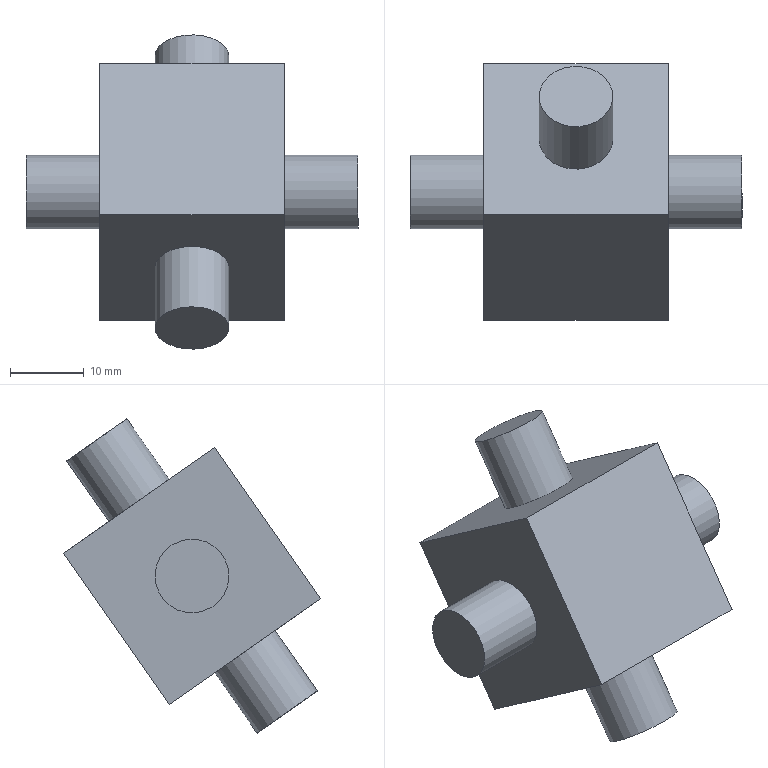Component | NX | UNIVERSAL_JOINT_CENTER_BLOCK_MODEL1 | 1 solid | 14 faces | box 45 x 34.82 x 42.6 mm | volume 18767 mm3 | plane 10 | cylinder 4 | commonest cylinder face diameters 10 x4
STEP:
#1=CARTESIAN_POINT('',(0.,0.,0.));
#2=DIRECTION('',(0.,0.,1.));
#3=DIRECTION('',(1.,0.,0.));
#4=AXIS2_PLACEMENT_3D('',#1,#2,#3);
#5=CARTESIAN_POINT('',(12.5,475.368,-241.274));
#6=VERTEX_POINT('',#5);
#7=CARTESIAN_POINT('',(12.5,461.028,-261.753));
#8=VERTEX_POINT('',#7);
#9=CARTESIAN_POINT('',(12.5,475.368,-241.274));
#10=DIRECTION('',(0.,-0.5736,-0.8192));
#11=VECTOR('',#10,1.);
#12=LINE('',#9,#11);
#13=CARTESIAN_POINT('',(-12.5,475.368,-241.274));
#14=DIRECTION('',(-0.,-0.8192,0.5736));
#15=DIRECTION('',(1.,-0.,0.));
#16=AXIS2_PLACEMENT_3D('',#13,#14,#15);
#17=PLANE('',#16);
#18=CARTESIAN_POINT('',(25.,-0.));
#19=DIRECTION('',(-0.,-1.));
#20=VECTOR('',#19,1.);
#21=LINE('',#18,#20);
#22=(GEOMETRIC_REPRESENTATION_CONTEXT(2)PARAMETRIC_REPRESENTATION_CONTEXT()REPRESENTATION_CONTEXT('',''));
#23=DEFINITIONAL_REPRESENTATION('',(#21),#22);
#24=PCURVE('',#17,#23);
#25=CARTESIAN_POINT('',(12.5,380.633,-190.2));
#26=DIRECTION('',(-1.,-0.,-0.));
#27=DIRECTION('',(-0.,-0.8192,0.5736));
#28=AXIS2_PLACEMENT_3D('',#25,#26,#27);
#29=PLANE('',#28);
#30=CARTESIAN_POINT('',(-106.897,12.5));
#31=DIRECTION('',(0.,-1.));
#32=VECTOR('',#31,1.);
#33=LINE('',#30,#32);
#34=(GEOMETRIC_REPRESENTATION_CONTEXT(2)PARAMETRIC_REPRESENTATION_CONTEXT()REPRESENTATION_CONTEXT('',''));
#35=DEFINITIONAL_REPRESENTATION('',(#33),#34);
#36=PCURVE('',#29,#35);
#37=SURFACE_CURVE('',#12,(#24,#36),.PCURVE_S1.);
#38=EDGE_CURVE('',#6,#8,#37,.T.);
#39=ORIENTED_EDGE('',*,*,#38,.T.);
#40=CARTESIAN_POINT('',(-12.5,461.028,-261.753));
#41=VERTEX_POINT('',#40);
#42=CARTESIAN_POINT('',(-12.5,461.028,-261.753));
#43=DIRECTION('',(1.,-0.,0.));
#44=VECTOR('',#43,1.);
#45=LINE('',#42,#44);
#46=CARTESIAN_POINT('',(-0.,-25.));
#47=DIRECTION('',(1.,0.));
#48=VECTOR('',#47,1.);
#49=LINE('',#46,#48);
#50=(GEOMETRIC_REPRESENTATION_CONTEXT(2)PARAMETRIC_REPRESENTATION_CONTEXT()REPRESENTATION_CONTEXT('',''));
#51=DEFINITIONAL_REPRESENTATION('',(#49),#50);
#52=PCURVE('',#17,#51);
#53=CARTESIAN_POINT('',(-12.5,461.028,-261.753));
#54=DIRECTION('',(0.,0.5736,0.8192));
#55=DIRECTION('',(0.866,-0.4096,0.2868));
#56=AXIS2_PLACEMENT_3D('',#53,#54,#55);
#57=PLANE('',#56);
#58=CARTESIAN_POINT('',(0.,0.));
#59=DIRECTION('',(0.866,0.5));
#60=VECTOR('',#59,1.);
#61=LINE('',#58,#60);
#62=(GEOMETRIC_REPRESENTATION_CONTEXT(2)PARAMETRIC_REPRESENTATION_CONTEXT()REPRESENTATION_CONTEXT('',''));
#63=DEFINITIONAL_REPRESENTATION('',(#61),#62);
#64=PCURVE('',#57,#63);
#65=SURFACE_CURVE('',#45,(#52,#64),.PCURVE_S1.);
#66=EDGE_CURVE('',#41,#8,#65,.T.);
#67=ORIENTED_EDGE('',*,*,#66,.F.);
#68=CARTESIAN_POINT('',(-12.5,475.368,-241.274));
#69=VERTEX_POINT('',#68);
#70=CARTESIAN_POINT('',(-12.5,475.368,-241.274));
#71=DIRECTION('',(0.,-0.5736,-0.8192));
#72=VECTOR('',#71,1.);
#73=LINE('',#70,#72);
#74=CARTESIAN_POINT('',(0.,0.));
#75=DIRECTION('',(-0.,-1.));
#76=VECTOR('',#75,1.);
#77=LINE('',#74,#76);
#78=(GEOMETRIC_REPRESENTATION_CONTEXT(2)PARAMETRIC_REPRESENTATION_CONTEXT()REPRESENTATION_CONTEXT('',''));
#79=DEFINITIONAL_REPRESENTATION('',(#77),#78);
#80=PCURVE('',#17,#79);
#81=CARTESIAN_POINT('',(-12.5,380.633,-190.2));
#82=DIRECTION('',(-1.,-0.,-0.));
#83=DIRECTION('',(-0.,-0.8192,0.5736));
#84=AXIS2_PLACEMENT_3D('',#81,#82,#83);
#85=PLANE('',#84);
#86=CARTESIAN_POINT('',(-106.897,12.5));
#87=DIRECTION('',(0.,-1.));
#88=VECTOR('',#87,1.);
#89=LINE('',#86,#88);
#90=(GEOMETRIC_REPRESENTATION_CONTEXT(2)PARAMETRIC_REPRESENTATION_CONTEXT()REPRESENTATION_CONTEXT('',''));
#91=DEFINITIONAL_REPRESENTATION('',(#89),#90);
#92=PCURVE('',#85,#91);
#93=SURFACE_CURVE('',#73,(#80,#92),.PCURVE_S1.);
#94=EDGE_CURVE('',#69,#41,#93,.T.);
#95=ORIENTED_EDGE('',*,*,#94,.F.);
#96=CARTESIAN_POINT('',(-12.5,475.368,-241.274));
#97=DIRECTION('',(1.,-0.,0.));
#98=VECTOR('',#97,1.);
#99=LINE('',#96,#98);
#100=CARTESIAN_POINT('',(0.,0.));
#101=DIRECTION('',(1.,0.));
#102=VECTOR('',#101,1.);
#103=LINE('',#100,#102);
#104=(GEOMETRIC_REPRESENTATION_CONTEXT(2)PARAMETRIC_REPRESENTATION_CONTEXT()REPRESENTATION_CONTEXT('',''));
#105=DEFINITIONAL_REPRESENTATION('',(#103),#104);
#106=PCURVE('',#17,#105);
#107=CARTESIAN_POINT('',(-12.5,454.889,-226.934));
#108=DIRECTION('',(0.,-0.5736,-0.8192));
#109=DIRECTION('',(-0.866,0.4096,-0.2868));
#110=AXIS2_PLACEMENT_3D('',#107,#108,#109);
#111=PLANE('',#110);
#112=CARTESIAN_POINT('',(12.5,21.651));
#113=DIRECTION('',(-0.866,0.5));
#114=VECTOR('',#113,1.);
#115=LINE('',#112,#114);
#116=(GEOMETRIC_REPRESENTATION_CONTEXT(2)PARAMETRIC_REPRESENTATION_CONTEXT()REPRESENTATION_CONTEXT('',''));
#117=DEFINITIONAL_REPRESENTATION('',(#115),#116);
#118=PCURVE('',#111,#117);
#119=SURFACE_CURVE('',#99,(#106,#118),.PCURVE_S1.);
#120=EDGE_CURVE('',#69,#6,#119,.T.);
#121=ORIENTED_EDGE('',*,*,#120,.T.);
#122=EDGE_LOOP('',(#39,#67,#95,#121));
#123=FACE_BOUND('',#122,.T.);
#124=ADVANCED_FACE('',(#123),#17,.F.);
#125=CARTESIAN_POINT('',(4.33,452.837,-256.017));
#126=VERTEX_POINT('',#125);
#127=CARTESIAN_POINT('',(0.,450.789,-254.583));
#128=DIRECTION('',(-0.,0.5736,0.8192));
#129=DIRECTION('',(0.866,0.4096,-0.2868));
#130=AXIS2_PLACEMENT_3D('',#127,#128,#129);
#131=CIRCLE('',#130,5.);
#132=CARTESIAN_POINT('',(17.075,-4.575));
#133=DIRECTION('',(0.5,0.866));
#134=AXIS2_PLACEMENT_2D('',#132,#133);
#135=CIRCLE('',#134,5.);
#136=(GEOMETRIC_REPRESENTATION_CONTEXT(2)PARAMETRIC_REPRESENTATION_CONTEXT()REPRESENTATION_CONTEXT('',''));
#137=DEFINITIONAL_REPRESENTATION('',(#135),#136);
#138=PCURVE('',#57,#137);
#139=CARTESIAN_POINT('',(0.,445.053,-262.774));
#140=DIRECTION('',(-0.,0.5736,0.8192));
#141=DIRECTION('',(0.866,-0.4096,0.2868));
#142=AXIS2_PLACEMENT_3D('',#139,#140,#141);
#143=CYLINDRICAL_SURFACE('',#142,5.);
#144=CARTESIAN_POINT('',(1.047,10.));
#145=DIRECTION('',(1.,0.));
#146=VECTOR('',#145,1.);
#147=LINE('',#144,#146);
#148=(GEOMETRIC_REPRESENTATION_CONTEXT(2)PARAMETRIC_REPRESENTATION_CONTEXT()REPRESENTATION_CONTEXT('',''));
#149=DEFINITIONAL_REPRESENTATION('',(#147),#148);
#150=PCURVE('',#143,#149);
#151=SURFACE_CURVE('',#131,(#138,#150),.PCURVE_S1.);
#152=EDGE_CURVE('',#126,#126,#151,.T.);
#153=ORIENTED_EDGE('',*,*,#152,.T.);
#154=EDGE_LOOP('',(#153));
#155=FACE_BOUND('',#154,.T.);
#156=CARTESIAN_POINT('',(12.5,440.55,-247.413));
#157=VERTEX_POINT('',#156);
#158=CARTESIAN_POINT('',(12.5,461.028,-261.753));
#159=DIRECTION('',(0.,-0.8192,0.5736));
#160=VECTOR('',#159,1.);
#161=LINE('',#158,#160);
#162=CARTESIAN_POINT('',(21.651,12.5));
#163=DIRECTION('',(0.5,-0.866));
#164=VECTOR('',#163,1.);
#165=LINE('',#162,#164);
#166=(GEOMETRIC_REPRESENTATION_CONTEXT(2)PARAMETRIC_REPRESENTATION_CONTEXT()REPRESENTATION_CONTEXT('',''));
#167=DEFINITIONAL_REPRESENTATION('',(#165),#166);
#168=PCURVE('',#57,#167);
#169=CARTESIAN_POINT('',(-106.897,-12.5));
#170=DIRECTION('',(1.,0.));
#171=VECTOR('',#170,1.);
#172=LINE('',#169,#171);
#173=(GEOMETRIC_REPRESENTATION_CONTEXT(2)PARAMETRIC_REPRESENTATION_CONTEXT()REPRESENTATION_CONTEXT('',''));
#174=DEFINITIONAL_REPRESENTATION('',(#172),#173);
#175=PCURVE('',#29,#174);
#176=SURFACE_CURVE('',#161,(#168,#175),.PCURVE_S1.);
#177=EDGE_CURVE('',#8,#157,#176,.T.);
#178=ORIENTED_EDGE('',*,*,#177,.T.);
#179=CARTESIAN_POINT('',(-12.5,440.55,-247.413));
#180=VERTEX_POINT('',#179);
#181=CARTESIAN_POINT('',(-12.5,440.55,-247.413));
#182=DIRECTION('',(1.,-0.,0.));
#183=VECTOR('',#182,1.);
#184=LINE('',#181,#183);
#185=CARTESIAN_POINT('',(12.5,-21.651));
#186=DIRECTION('',(0.866,0.5));
#187=VECTOR('',#186,1.);
#188=LINE('',#185,#187);
#189=(GEOMETRIC_REPRESENTATION_CONTEXT(2)PARAMETRIC_REPRESENTATION_CONTEXT()REPRESENTATION_CONTEXT('',''));
#190=DEFINITIONAL_REPRESENTATION('',(#188),#189);
#191=PCURVE('',#57,#190);
#192=CARTESIAN_POINT('',(-12.5,440.55,-247.413));
#193=DIRECTION('',(0.,0.8192,-0.5736));
#194=DIRECTION('',(-1.,0.,-0.));
#195=AXIS2_PLACEMENT_3D('',#192,#193,#194);
#196=PLANE('',#195);
#197=CARTESIAN_POINT('',(0.,0.));
#198=DIRECTION('',(-1.,0.));
#199=VECTOR('',#198,1.);
#200=LINE('',#197,#199);
#201=(GEOMETRIC_REPRESENTATION_CONTEXT(2)PARAMETRIC_REPRESENTATION_CONTEXT()REPRESENTATION_CONTEXT('',''));
#202=DEFINITIONAL_REPRESENTATION('',(#200),#201);
#203=PCURVE('',#196,#202);
#204=SURFACE_CURVE('',#184,(#191,#203),.PCURVE_S1.);
#205=EDGE_CURVE('',#180,#157,#204,.T.);
#206=ORIENTED_EDGE('',*,*,#205,.F.);
#207=CARTESIAN_POINT('',(-12.5,461.028,-261.753));
#208=DIRECTION('',(0.,-0.8192,0.5736));
#209=VECTOR('',#208,1.);
#210=LINE('',#207,#209);
#211=CARTESIAN_POINT('',(0.,0.));
#212=DIRECTION('',(0.5,-0.866));
#213=VECTOR('',#212,1.);
#214=LINE('',#211,#213);
#215=(GEOMETRIC_REPRESENTATION_CONTEXT(2)PARAMETRIC_REPRESENTATION_CONTEXT()REPRESENTATION_CONTEXT('',''));
#216=DEFINITIONAL_REPRESENTATION('',(#214),#215);
#217=PCURVE('',#57,#216);
#218=CARTESIAN_POINT('',(-106.897,-12.5));
#219=DIRECTION('',(1.,0.));
#220=VECTOR('',#219,1.);
#221=LINE('',#218,#220);
#222=(GEOMETRIC_REPRESENTATION_CONTEXT(2)PARAMETRIC_REPRESENTATION_CONTEXT()REPRESENTATION_CONTEXT('',''));
#223=DEFINITIONAL_REPRESENTATION('',(#221),#222);
#224=PCURVE('',#85,#223);
#225=SURFACE_CURVE('',#210,(#217,#224),.PCURVE_S1.);
#226=EDGE_CURVE('',#41,#180,#225,.T.);
#227=ORIENTED_EDGE('',*,*,#226,.F.);
#228=ORIENTED_EDGE('',*,*,#66,.T.);
#229=EDGE_LOOP('',(#178,#206,#227,#228));
#230=FACE_BOUND('',#229,.T.);
#231=ADVANCED_FACE('',(#155,#230),#57,.F.);
#232=CARTESIAN_POINT('',(12.5,454.889,-226.934));
#233=VERTEX_POINT('',#232);
#234=CARTESIAN_POINT('',(12.5,440.55,-247.413));
#235=DIRECTION('',(0.,0.5736,0.8192));
#236=VECTOR('',#235,1.);
#237=LINE('',#234,#236);
#238=CARTESIAN_POINT('',(-25.,-0.));
#239=DIRECTION('',(-0.,1.));
#240=VECTOR('',#239,1.);
#241=LINE('',#238,#240);
#242=(GEOMETRIC_REPRESENTATION_CONTEXT(2)PARAMETRIC_REPRESENTATION_CONTEXT()REPRESENTATION_CONTEXT('',''));
#243=DEFINITIONAL_REPRESENTATION('',(#241),#242);
#244=PCURVE('',#196,#243);
#245=CARTESIAN_POINT('',(-81.897,-12.5));
#246=DIRECTION('',(0.,1.));
#247=VECTOR('',#246,1.);
#248=LINE('',#245,#247);
#249=(GEOMETRIC_REPRESENTATION_CONTEXT(2)PARAMETRIC_REPRESENTATION_CONTEXT()REPRESENTATION_CONTEXT('',''));
#250=DEFINITIONAL_REPRESENTATION('',(#248),#249);
#251=PCURVE('',#29,#250);
#252=SURFACE_CURVE('',#237,(#244,#251),.PCURVE_S1.);
#253=EDGE_CURVE('',#157,#233,#252,.T.);
#254=ORIENTED_EDGE('',*,*,#253,.T.);
#255=CARTESIAN_POINT('',(-12.5,454.889,-226.934));
#256=VERTEX_POINT('',#255);
#257=CARTESIAN_POINT('',(-12.5,454.889,-226.934));
#258=DIRECTION('',(1.,-0.,0.));
#259=VECTOR('',#258,1.);
#260=LINE('',#257,#259);
#261=CARTESIAN_POINT('',(-0.,25.));
#262=DIRECTION('',(-1.,0.));
#263=VECTOR('',#262,1.);
#264=LINE('',#261,#263);
#265=(GEOMETRIC_REPRESENTATION_CONTEXT(2)PARAMETRIC_REPRESENTATION_CONTEXT()REPRESENTATION_CONTEXT('',''));
#266=DEFINITIONAL_REPRESENTATION('',(#264),#265);
#267=PCURVE('',#196,#266);
#268=CARTESIAN_POINT('',(0.,0.));
#269=DIRECTION('',(-0.866,0.5));
#270=VECTOR('',#269,1.);
#271=LINE('',#268,#270);
#272=(GEOMETRIC_REPRESENTATION_CONTEXT(2)PARAMETRIC_REPRESENTATION_CONTEXT()REPRESENTATION_CONTEXT('',''));
#273=DEFINITIONAL_REPRESENTATION('',(#271),#272);
#274=PCURVE('',#111,#273);
#275=SURFACE_CURVE('',#260,(#267,#274),.PCURVE_S1.);
#276=EDGE_CURVE('',#256,#233,#275,.T.);
#277=ORIENTED_EDGE('',*,*,#276,.F.);
#278=CARTESIAN_POINT('',(-12.5,440.55,-247.413));
#279=DIRECTION('',(0.,0.5736,0.8192));
#280=VECTOR('',#279,1.);
#281=LINE('',#278,#280);
#282=CARTESIAN_POINT('',(0.,0.));
#283=DIRECTION('',(-0.,1.));
#284=VECTOR('',#283,1.);
#285=LINE('',#282,#284);
#286=(GEOMETRIC_REPRESENTATION_CONTEXT(2)PARAMETRIC_REPRESENTATION_CONTEXT()REPRESENTATION_CONTEXT('',''));
#287=DEFINITIONAL_REPRESENTATION('',(#285),#286);
#288=PCURVE('',#196,#287);
#289=CARTESIAN_POINT('',(-81.897,-12.5));
#290=DIRECTION('',(0.,1.));
#291=VECTOR('',#290,1.);
#292=LINE('',#289,#291);
#293=(GEOMETRIC_REPRESENTATION_CONTEXT(2)PARAMETRIC_REPRESENTATION_CONTEXT()REPRESENTATION_CONTEXT('',''));
#294=DEFINITIONAL_REPRESENTATION('',(#292),#293);
#295=PCURVE('',#85,#294);
#296=SURFACE_CURVE('',#281,(#288,#295),.PCURVE_S1.);
#297=EDGE_CURVE('',#180,#256,#296,.T.);
#298=ORIENTED_EDGE('',*,*,#297,.F.);
#299=ORIENTED_EDGE('',*,*,#205,.T.);
#300=EDGE_LOOP('',(#254,#277,#298,#299));
#301=FACE_BOUND('',#300,.T.);
#302=ADVANCED_FACE('',(#301),#196,.F.);
#303=CARTESIAN_POINT('',(-4.33,467.176,-235.538));
#304=VERTEX_POINT('',#303);
#305=CARTESIAN_POINT('',(0.,465.128,-234.104));
#306=DIRECTION('',(0.,-0.5736,-0.8192));
#307=DIRECTION('',(-0.866,0.4096,-0.2868));
#308=AXIS2_PLACEMENT_3D('',#305,#306,#307);
#309=CIRCLE('',#308,5.);
#310=CARTESIAN_POINT('',(-4.575,17.075));
#311=DIRECTION('',(1.,0.));
#312=AXIS2_PLACEMENT_2D('',#310,#311);
#313=CIRCLE('',#312,5.);
#314=(GEOMETRIC_REPRESENTATION_CONTEXT(2)PARAMETRIC_REPRESENTATION_CONTEXT()REPRESENTATION_CONTEXT('',''));
#315=DEFINITIONAL_REPRESENTATION('',(#313),#314);
#316=PCURVE('',#111,#315);
#317=CARTESIAN_POINT('',(0.,470.864,-225.913));
#318=DIRECTION('',(0.,-0.5736,-0.8192));
#319=DIRECTION('',(-0.866,0.4096,-0.2868));
#320=AXIS2_PLACEMENT_3D('',#317,#318,#319);
#321=CYLINDRICAL_SURFACE('',#320,5.);
#322=CARTESIAN_POINT('',(0.,10.));
#323=DIRECTION('',(1.,0.));
#324=VECTOR('',#323,1.);
#325=LINE('',#322,#324);
#326=(GEOMETRIC_REPRESENTATION_CONTEXT(2)PARAMETRIC_REPRESENTATION_CONTEXT()REPRESENTATION_CONTEXT('',''));
#327=DEFINITIONAL_REPRESENTATION('',(#325),#326);
#328=PCURVE('',#321,#327);
#329=SURFACE_CURVE('',#309,(#316,#328),.PCURVE_S1.);
#330=EDGE_CURVE('',#304,#304,#329,.T.);
#331=ORIENTED_EDGE('',*,*,#330,.T.);
#332=EDGE_LOOP('',(#331));
#333=FACE_BOUND('',#332,.T.);
#334=CARTESIAN_POINT('',(12.5,454.889,-226.934));
#335=DIRECTION('',(0.,0.8192,-0.5736));
#336=VECTOR('',#335,1.);
#337=LINE('',#334,#336);
#338=CARTESIAN_POINT('',(-21.651,12.5));
#339=DIRECTION('',(0.5,0.866));
#340=VECTOR('',#339,1.);
#341=LINE('',#338,#340);
#342=(GEOMETRIC_REPRESENTATION_CONTEXT(2)PARAMETRIC_REPRESENTATION_CONTEXT()REPRESENTATION_CONTEXT('',''));
#343=DEFINITIONAL_REPRESENTATION('',(#341),#342);
#344=PCURVE('',#111,#343);
#345=CARTESIAN_POINT('',(-81.897,12.5));
#346=DIRECTION('',(-1.,0.));
#347=VECTOR('',#346,1.);
#348=LINE('',#345,#347);
#349=(GEOMETRIC_REPRESENTATION_CONTEXT(2)PARAMETRIC_REPRESENTATION_CONTEXT()REPRESENTATION_CONTEXT('',''));
#350=DEFINITIONAL_REPRESENTATION('',(#348),#349);
#351=PCURVE('',#29,#350);
#352=SURFACE_CURVE('',#337,(#344,#351),.PCURVE_S1.);
#353=EDGE_CURVE('',#233,#6,#352,.T.);
#354=ORIENTED_EDGE('',*,*,#353,.T.);
#355=ORIENTED_EDGE('',*,*,#120,.F.);
#356=CARTESIAN_POINT('',(-12.5,454.889,-226.934));
#357=DIRECTION('',(0.,0.8192,-0.5736));
#358=VECTOR('',#357,1.);
#359=LINE('',#356,#358);
#360=CARTESIAN_POINT('',(0.,0.));
#361=DIRECTION('',(0.5,0.866));
#362=VECTOR('',#361,1.);
#363=LINE('',#360,#362);
#364=(GEOMETRIC_REPRESENTATION_CONTEXT(2)PARAMETRIC_REPRESENTATION_CONTEXT()REPRESENTATION_CONTEXT('',''));
#365=DEFINITIONAL_REPRESENTATION('',(#363),#364);
#366=PCURVE('',#111,#365);
#367=CARTESIAN_POINT('',(-81.897,12.5));
#368=DIRECTION('',(-1.,0.));
#369=VECTOR('',#368,1.);
#370=LINE('',#367,#369);
#371=(GEOMETRIC_REPRESENTATION_CONTEXT(2)PARAMETRIC_REPRESENTATION_CONTEXT()REPRESENTATION_CONTEXT('',''));
#372=DEFINITIONAL_REPRESENTATION('',(#370),#371);
#373=PCURVE('',#85,#372);
#374=SURFACE_CURVE('',#359,(#366,#373),.PCURVE_S1.);
#375=EDGE_CURVE('',#256,#69,#374,.T.);
#376=ORIENTED_EDGE('',*,*,#375,.F.);
#377=ORIENTED_EDGE('',*,*,#276,.T.);
#378=EDGE_LOOP('',(#354,#355,#376,#377));
#379=FACE_BOUND('',#378,.T.);
#380=ADVANCED_FACE('',(#333,#379),#111,.F.);
#381=CARTESIAN_POINT('',(-12.5,457.523,-249.325));
#382=VERTEX_POINT('',#381);
#383=CARTESIAN_POINT('',(-12.5,457.959,-244.344));
#384=DIRECTION('',(1.,0.,0.));
#385=DIRECTION('',(0.,-0.08716,-0.9962));
#386=AXIS2_PLACEMENT_3D('',#383,#384,#385);
#387=CIRCLE('',#386,5.);
#388=CARTESIAN_POINT('',(-96.897,-4.33));
#389=CARTESIAN_POINT('',(-104.397,-0.));
#390=CARTESIAN_POINT('',(-96.897,4.33));
#391=CARTESIAN_POINT('',(-89.397,8.66));
#392=CARTESIAN_POINT('',(-89.397,-0.));
#393=CARTESIAN_POINT('',(-89.397,-8.66));
#394=CARTESIAN_POINT('',(-96.897,-4.33));
#395=(BOUNDED_CURVE()B_SPLINE_CURVE(2,(#388,#389,#390,#391,#392,#393,#394),.UNSPECIFIED.,.T.,.F.)B_SPLINE_CURVE_WITH_KNOTS((1,2,2,2,2,1),(-2.094,0.,2.094,4.189,6.283,8.378),.UNSPECIFIED.)CURVE()GEOMETRIC_REPRESENTATION_ITEM()RATIONAL_B_SPLINE_CURVE((1.,0.5,1.,0.5,1.,0.5,1.))REPRESENTATION_ITEM(''));
#396=(GEOMETRIC_REPRESENTATION_CONTEXT(2)PARAMETRIC_REPRESENTATION_CONTEXT()REPRESENTATION_CONTEXT('',''));
#397=DEFINITIONAL_REPRESENTATION('',(#395),#396);
#398=PCURVE('',#85,#397);
#399=CARTESIAN_POINT('',(-22.5,457.959,-244.344));
#400=DIRECTION('',(1.,0.,0.));
#401=DIRECTION('',(0.,0.8192,-0.5736));
#402=AXIS2_PLACEMENT_3D('',#399,#400,#401);
#403=CYLINDRICAL_SURFACE('',#402,5.);
#404=CARTESIAN_POINT('',(5.236,10.));
#405=DIRECTION('',(1.,0.));
#406=VECTOR('',#405,1.);
#407=LINE('',#404,#406);
#408=(GEOMETRIC_REPRESENTATION_CONTEXT(2)PARAMETRIC_REPRESENTATION_CONTEXT()REPRESENTATION_CONTEXT('',''));
#409=DEFINITIONAL_REPRESENTATION('',(#407),#408);
#410=PCURVE('',#403,#409);
#411=SURFACE_CURVE('',#387,(#398,#410),.PCURVE_S1.);
#412=EDGE_CURVE('',#382,#382,#411,.T.);
#413=ORIENTED_EDGE('',*,*,#412,.T.);
#414=EDGE_LOOP('',(#413));
#415=FACE_BOUND('',#414,.T.);
#416=ORIENTED_EDGE('',*,*,#94,.T.);
#417=ORIENTED_EDGE('',*,*,#226,.T.);
#418=ORIENTED_EDGE('',*,*,#297,.T.);
#419=ORIENTED_EDGE('',*,*,#375,.T.);
#420=EDGE_LOOP('',(#416,#417,#418,#419));
#421=FACE_BOUND('',#420,.T.);
#422=ADVANCED_FACE('',(#415,#421),#85,.T.);
#423=CARTESIAN_POINT('',(12.5,462.49,-242.23));
#424=VERTEX_POINT('',#423);
#425=CARTESIAN_POINT('',(12.5,457.959,-244.344));
#426=DIRECTION('',(-1.,-0.,-0.));
#427=DIRECTION('',(-0.,0.9063,0.4226));
#428=AXIS2_PLACEMENT_3D('',#425,#426,#427);
#429=CIRCLE('',#428,5.);
#430=CARTESIAN_POINT('',(-94.397,-0.));
#431=DIRECTION('',(-0.5,0.866));
#432=AXIS2_PLACEMENT_2D('',#430,#431);
#433=CIRCLE('',#432,5.);
#434=(GEOMETRIC_REPRESENTATION_CONTEXT(2)PARAMETRIC_REPRESENTATION_CONTEXT()REPRESENTATION_CONTEXT('',''));
#435=DEFINITIONAL_REPRESENTATION('',(#433),#434);
#436=PCURVE('',#29,#435);
#437=CARTESIAN_POINT('',(22.5,457.959,-244.344));
#438=DIRECTION('',(-1.,-0.,-0.));
#439=DIRECTION('',(-0.,-0.8192,0.5736));
#440=AXIS2_PLACEMENT_3D('',#437,#438,#439);
#441=CYLINDRICAL_SURFACE('',#440,5.);
#442=CARTESIAN_POINT('',(2.094,10.));
#443=DIRECTION('',(1.,0.));
#444=VECTOR('',#443,1.);
#445=LINE('',#442,#444);
#446=(GEOMETRIC_REPRESENTATION_CONTEXT(2)PARAMETRIC_REPRESENTATION_CONTEXT()REPRESENTATION_CONTEXT('',''));
#447=DEFINITIONAL_REPRESENTATION('',(#445),#446);
#448=PCURVE('',#441,#447);
#449=SURFACE_CURVE('',#429,(#436,#448),.PCURVE_S1.);
#450=EDGE_CURVE('',#424,#424,#449,.T.);
#451=ORIENTED_EDGE('',*,*,#450,.T.);
#452=EDGE_LOOP('',(#451));
#453=FACE_BOUND('',#452,.T.);
#454=ORIENTED_EDGE('',*,*,#38,.F.);
#455=ORIENTED_EDGE('',*,*,#353,.F.);
#456=ORIENTED_EDGE('',*,*,#253,.F.);
#457=ORIENTED_EDGE('',*,*,#177,.F.);
#458=EDGE_LOOP('',(#454,#455,#456,#457));
#459=FACE_BOUND('',#458,.T.);
#460=ADVANCED_FACE('',(#453,#459),#29,.F.);
#461=CARTESIAN_POINT('',(-4.33,472.912,-227.347));
#462=VERTEX_POINT('',#461);
#463=CARTESIAN_POINT('',(0.,470.864,-225.913));
#464=DIRECTION('',(0.,-0.5736,-0.8192));
#465=DIRECTION('',(-0.866,0.4096,-0.2868));
#466=AXIS2_PLACEMENT_3D('',#463,#464,#465);
#467=CIRCLE('',#466,5.);
#468=CARTESIAN_POINT('',(0.,-0.));
#469=DIRECTION('',(1.,0.));
#470=VECTOR('',#469,1.);
#471=LINE('',#468,#470);
#472=(GEOMETRIC_REPRESENTATION_CONTEXT(2)PARAMETRIC_REPRESENTATION_CONTEXT()REPRESENTATION_CONTEXT('',''));
#473=DEFINITIONAL_REPRESENTATION('',(#471),#472);
#474=PCURVE('',#321,#473);
#475=CARTESIAN_POINT('',(0.,470.864,-225.913));
#476=DIRECTION('',(0.,-0.5736,-0.8192));
#477=DIRECTION('',(-0.866,0.4096,-0.2868));
#478=AXIS2_PLACEMENT_3D('',#475,#476,#477);
#479=PLANE('',#478);
#480=CARTESIAN_POINT('',(0.,0.));
#481=DIRECTION('',(1.,0.));
#482=AXIS2_PLACEMENT_2D('',#480,#481);
#483=CIRCLE('',#482,5.);
#484=(GEOMETRIC_REPRESENTATION_CONTEXT(2)PARAMETRIC_REPRESENTATION_CONTEXT()REPRESENTATION_CONTEXT('',''));
#485=DEFINITIONAL_REPRESENTATION('',(#483),#484);
#486=PCURVE('',#479,#485);
#487=SURFACE_CURVE('',#467,(#474,#486),.PCURVE_S1.);
#488=EDGE_CURVE('',#462,#462,#487,.T.);
#489=ORIENTED_EDGE('',*,*,#488,.T.);
#490=CARTESIAN_POINT('',(-4.33,472.912,-227.347));
#491=CARTESIAN_POINT('',(-4.33,467.176,-235.538));
#492=B_SPLINE_CURVE_WITH_KNOTS('',1,(#490,#491),.UNSPECIFIED.,.F.,.F.,(2,2),(-0.,10.),.PIECEWISE_BEZIER_KNOTS.);
#493=CARTESIAN_POINT('',(6.283,0.));
#494=DIRECTION('',(0.,1.));
#495=VECTOR('',#494,1.);
#496=LINE('',#493,#495);
#497=(GEOMETRIC_REPRESENTATION_CONTEXT(2)PARAMETRIC_REPRESENTATION_CONTEXT()REPRESENTATION_CONTEXT('',''));
#498=DEFINITIONAL_REPRESENTATION('',(#496),#497);
#499=PCURVE('',#321,#498);
#500=CARTESIAN_POINT('',(0.,0.));
#501=DIRECTION('',(0.,1.));
#502=VECTOR('',#501,1.);
#503=LINE('',#500,#502);
#504=(GEOMETRIC_REPRESENTATION_CONTEXT(2)PARAMETRIC_REPRESENTATION_CONTEXT()REPRESENTATION_CONTEXT('',''));
#505=DEFINITIONAL_REPRESENTATION('',(#503),#504);
#506=PCURVE('',#321,#505);
#507=SEAM_CURVE('',#492,(#499,#506),.PCURVE_S1.);
#508=EDGE_CURVE('',#462,#304,#507,.T.);
#509=ORIENTED_EDGE('',*,*,#508,.T.);
#510=ORIENTED_EDGE('',*,*,#330,.F.);
#511=ORIENTED_EDGE('',*,*,#508,.F.);
#512=EDGE_LOOP('',(#489,#509,#510,#511));
#513=FACE_BOUND('',#512,.T.);
#514=ADVANCED_FACE('',(#513),#321,.T.);
#515=ORIENTED_EDGE('',*,*,#488,.F.);
#516=EDGE_LOOP('',(#515));
#517=FACE_BOUND('',#516,.T.);
#518=ADVANCED_FACE('',(#517),#479,.F.);
#519=CARTESIAN_POINT('',(22.5,462.49,-242.23));
#520=VERTEX_POINT('',#519);
#521=CARTESIAN_POINT('',(22.5,457.959,-244.344));
#522=DIRECTION('',(-1.,-0.,-0.));
#523=DIRECTION('',(-0.,0.9063,0.4226));
#524=AXIS2_PLACEMENT_3D('',#521,#522,#523);
#525=CIRCLE('',#524,5.);
#526=CARTESIAN_POINT('',(2.094,0.));
#527=DIRECTION('',(1.,0.));
#528=VECTOR('',#527,1.);
#529=LINE('',#526,#528);
#530=(GEOMETRIC_REPRESENTATION_CONTEXT(2)PARAMETRIC_REPRESENTATION_CONTEXT()REPRESENTATION_CONTEXT('',''));
#531=DEFINITIONAL_REPRESENTATION('',(#529),#530);
#532=PCURVE('',#441,#531);
#533=CARTESIAN_POINT('',(22.5,457.959,-244.344));
#534=DIRECTION('',(-1.,-0.,-0.));
#535=DIRECTION('',(-0.,-0.8192,0.5736));
#536=AXIS2_PLACEMENT_3D('',#533,#534,#535);
#537=PLANE('',#536);
#538=CARTESIAN_POINT('',(0.,0.));
#539=DIRECTION('',(-0.5,0.866));
#540=AXIS2_PLACEMENT_2D('',#538,#539);
#541=CIRCLE('',#540,5.);
#542=(GEOMETRIC_REPRESENTATION_CONTEXT(2)PARAMETRIC_REPRESENTATION_CONTEXT()REPRESENTATION_CONTEXT('',''));
#543=DEFINITIONAL_REPRESENTATION('',(#541),#542);
#544=PCURVE('',#537,#543);
#545=SURFACE_CURVE('',#525,(#532,#544),.PCURVE_S1.);
#546=EDGE_CURVE('',#520,#520,#545,.T.);
#547=ORIENTED_EDGE('',*,*,#546,.T.);
#548=CARTESIAN_POINT('',(22.5,462.49,-242.23));
#549=CARTESIAN_POINT('',(12.5,462.49,-242.23));
#550=B_SPLINE_CURVE_WITH_KNOTS('',1,(#548,#549),.UNSPECIFIED.,.F.,.F.,(2,2),(0.,10.),.PIECEWISE_BEZIER_KNOTS.);
#551=CARTESIAN_POINT('',(8.378,0.));
#552=DIRECTION('',(0.,1.));
#553=VECTOR('',#552,1.);
#554=LINE('',#551,#553);
#555=(GEOMETRIC_REPRESENTATION_CONTEXT(2)PARAMETRIC_REPRESENTATION_CONTEXT()REPRESENTATION_CONTEXT('',''));
#556=DEFINITIONAL_REPRESENTATION('',(#554),#555);
#557=PCURVE('',#441,#556);
#558=CARTESIAN_POINT('',(2.094,0.));
#559=DIRECTION('',(0.,1.));
#560=VECTOR('',#559,1.);
#561=LINE('',#558,#560);
#562=(GEOMETRIC_REPRESENTATION_CONTEXT(2)PARAMETRIC_REPRESENTATION_CONTEXT()REPRESENTATION_CONTEXT('',''));
#563=DEFINITIONAL_REPRESENTATION('',(#561),#562);
#564=PCURVE('',#441,#563);
#565=SEAM_CURVE('',#550,(#557,#564),.PCURVE_S1.);
#566=EDGE_CURVE('',#520,#424,#565,.T.);
#567=ORIENTED_EDGE('',*,*,#566,.T.);
#568=ORIENTED_EDGE('',*,*,#450,.F.);
#569=ORIENTED_EDGE('',*,*,#566,.F.);
#570=EDGE_LOOP('',(#547,#567,#568,#569));
#571=FACE_BOUND('',#570,.T.);
#572=ADVANCED_FACE('',(#571),#441,.T.);
#573=ORIENTED_EDGE('',*,*,#546,.F.);
#574=EDGE_LOOP('',(#573));
#575=FACE_BOUND('',#574,.T.);
#576=ADVANCED_FACE('',(#575),#537,.F.);
#577=CARTESIAN_POINT('',(4.33,447.101,-264.208));
#578=VERTEX_POINT('',#577);
#579=CARTESIAN_POINT('',(0.,445.053,-262.774));
#580=DIRECTION('',(-0.,0.5736,0.8192));
#581=DIRECTION('',(0.866,0.4096,-0.2868));
#582=AXIS2_PLACEMENT_3D('',#579,#580,#581);
#583=CIRCLE('',#582,5.);
#584=CARTESIAN_POINT('',(1.047,0.));
#585=DIRECTION('',(1.,0.));
#586=VECTOR('',#585,1.);
#587=LINE('',#584,#586);
#588=(GEOMETRIC_REPRESENTATION_CONTEXT(2)PARAMETRIC_REPRESENTATION_CONTEXT()REPRESENTATION_CONTEXT('',''));
#589=DEFINITIONAL_REPRESENTATION('',(#587),#588);
#590=PCURVE('',#143,#589);
#591=CARTESIAN_POINT('',(0.,445.053,-262.774));
#592=DIRECTION('',(-0.,0.5736,0.8192));
#593=DIRECTION('',(0.866,-0.4096,0.2868));
#594=AXIS2_PLACEMENT_3D('',#591,#592,#593);
#595=PLANE('',#594);
#596=CARTESIAN_POINT('',(0.,0.));
#597=DIRECTION('',(0.5,0.866));
#598=AXIS2_PLACEMENT_2D('',#596,#597);
#599=CIRCLE('',#598,5.);
#600=(GEOMETRIC_REPRESENTATION_CONTEXT(2)PARAMETRIC_REPRESENTATION_CONTEXT()REPRESENTATION_CONTEXT('',''));
#601=DEFINITIONAL_REPRESENTATION('',(#599),#600);
#602=PCURVE('',#595,#601);
#603=SURFACE_CURVE('',#583,(#590,#602),.PCURVE_S1.);
#604=EDGE_CURVE('',#578,#578,#603,.T.);
#605=ORIENTED_EDGE('',*,*,#604,.T.);
#606=CARTESIAN_POINT('',(4.33,447.101,-264.208));
#607=CARTESIAN_POINT('',(4.33,452.837,-256.017));
#608=B_SPLINE_CURVE_WITH_KNOTS('',1,(#606,#607),.UNSPECIFIED.,.F.,.F.,(2,2),(0.,10.),.PIECEWISE_BEZIER_KNOTS.);
#609=CARTESIAN_POINT('',(7.33,0.));
#610=DIRECTION('',(0.,1.));
#611=VECTOR('',#610,1.);
#612=LINE('',#609,#611);
#613=(GEOMETRIC_REPRESENTATION_CONTEXT(2)PARAMETRIC_REPRESENTATION_CONTEXT()REPRESENTATION_CONTEXT('',''));
#614=DEFINITIONAL_REPRESENTATION('',(#612),#613);
#615=PCURVE('',#143,#614);
#616=CARTESIAN_POINT('',(1.047,0.));
#617=DIRECTION('',(0.,1.));
#618=VECTOR('',#617,1.);
#619=LINE('',#616,#618);
#620=(GEOMETRIC_REPRESENTATION_CONTEXT(2)PARAMETRIC_REPRESENTATION_CONTEXT()REPRESENTATION_CONTEXT('',''));
#621=DEFINITIONAL_REPRESENTATION('',(#619),#620);
#622=PCURVE('',#143,#621);
#623=SEAM_CURVE('',#608,(#615,#622),.PCURVE_S1.);
#624=EDGE_CURVE('',#578,#126,#623,.T.);
#625=ORIENTED_EDGE('',*,*,#624,.T.);
#626=ORIENTED_EDGE('',*,*,#152,.F.);
#627=ORIENTED_EDGE('',*,*,#624,.F.);
#628=EDGE_LOOP('',(#605,#625,#626,#627));
#629=FACE_BOUND('',#628,.T.);
#630=ADVANCED_FACE('',(#629),#143,.T.);
#631=ORIENTED_EDGE('',*,*,#604,.F.);
#632=EDGE_LOOP('',(#631));
#633=FACE_BOUND('',#632,.T.);
#634=ADVANCED_FACE('',(#633),#595,.F.);
#635=CARTESIAN_POINT('',(-22.5,457.523,-249.325));
#636=VERTEX_POINT('',#635);
#637=CARTESIAN_POINT('',(-22.5,457.959,-244.344));
#638=DIRECTION('',(1.,0.,0.));
#639=DIRECTION('',(0.,-0.08716,-0.9962));
#640=AXIS2_PLACEMENT_3D('',#637,#638,#639);
#641=CIRCLE('',#640,5.);
#642=CARTESIAN_POINT('',(5.236,0.));
#643=DIRECTION('',(1.,0.));
#644=VECTOR('',#643,1.);
#645=LINE('',#642,#644);
#646=(GEOMETRIC_REPRESENTATION_CONTEXT(2)PARAMETRIC_REPRESENTATION_CONTEXT()REPRESENTATION_CONTEXT('',''));
#647=DEFINITIONAL_REPRESENTATION('',(#645),#646);
#648=PCURVE('',#403,#647);
#649=CARTESIAN_POINT('',(-22.5,457.959,-244.344));
#650=DIRECTION('',(1.,0.,0.));
#651=DIRECTION('',(0.,0.8192,-0.5736));
#652=AXIS2_PLACEMENT_3D('',#649,#650,#651);
#653=PLANE('',#652);
#654=CARTESIAN_POINT('',(0.,0.));
#655=DIRECTION('',(0.5,-0.866));
#656=AXIS2_PLACEMENT_2D('',#654,#655);
#657=CIRCLE('',#656,5.);
#658=(GEOMETRIC_REPRESENTATION_CONTEXT(2)PARAMETRIC_REPRESENTATION_CONTEXT()REPRESENTATION_CONTEXT('',''));
#659=DEFINITIONAL_REPRESENTATION('',(#657),#658);
#660=PCURVE('',#653,#659);
#661=SURFACE_CURVE('',#641,(#648,#660),.PCURVE_S1.);
#662=EDGE_CURVE('',#636,#636,#661,.T.);
#663=ORIENTED_EDGE('',*,*,#662,.T.);
#664=CARTESIAN_POINT('',(-22.5,457.523,-249.325));
#665=CARTESIAN_POINT('',(-12.5,457.523,-249.325));
#666=B_SPLINE_CURVE_WITH_KNOTS('',1,(#664,#665),.UNSPECIFIED.,.F.,.F.,(2,2),(0.,10.),.PIECEWISE_BEZIER_KNOTS.);
#667=CARTESIAN_POINT('',(11.519,0.));
#668=DIRECTION('',(0.,1.));
#669=VECTOR('',#668,1.);
#670=LINE('',#667,#669);
#671=(GEOMETRIC_REPRESENTATION_CONTEXT(2)PARAMETRIC_REPRESENTATION_CONTEXT()REPRESENTATION_CONTEXT('',''));
#672=DEFINITIONAL_REPRESENTATION('',(#670),#671);
#673=PCURVE('',#403,#672);
#674=CARTESIAN_POINT('',(5.236,0.));
#675=DIRECTION('',(0.,1.));
#676=VECTOR('',#675,1.);
#677=LINE('',#674,#676);
#678=(GEOMETRIC_REPRESENTATION_CONTEXT(2)PARAMETRIC_REPRESENTATION_CONTEXT()REPRESENTATION_CONTEXT('',''));
#679=DEFINITIONAL_REPRESENTATION('',(#677),#678);
#680=PCURVE('',#403,#679);
#681=SEAM_CURVE('',#666,(#673,#680),.PCURVE_S1.);
#682=EDGE_CURVE('',#636,#382,#681,.T.);
#683=ORIENTED_EDGE('',*,*,#682,.T.);
#684=ORIENTED_EDGE('',*,*,#412,.F.);
#685=ORIENTED_EDGE('',*,*,#682,.F.);
#686=EDGE_LOOP('',(#663,#683,#684,#685));
#687=FACE_BOUND('',#686,.T.);
#688=ADVANCED_FACE('',(#687),#403,.T.);
#689=ORIENTED_EDGE('',*,*,#662,.F.);
#690=EDGE_LOOP('',(#689));
#691=FACE_BOUND('',#690,.T.);
#692=ADVANCED_FACE('',(#691),#653,.F.);
#693=CLOSED_SHELL('',(#124,#231,#302,#380,#422,#460,#514,#518,#572,#576,#630,#634,#688,#692));
#694=MANIFOLD_SOLID_BREP('',#693);
#695=(LENGTH_UNIT()NAMED_UNIT(*)SI_UNIT(.MILLI.,.METRE.));
#696=UNCERTAINTY_MEASURE_WITH_UNIT(LENGTH_MEASURE(0.000005),#695,'','');
#697=(NAMED_UNIT(*)PLANE_ANGLE_UNIT()SI_UNIT($,.RADIAN.));
#698=(NAMED_UNIT(*)SI_UNIT($,.STERADIAN.)SOLID_ANGLE_UNIT());
#699=(GEOMETRIC_REPRESENTATION_CONTEXT(3)GLOBAL_UNCERTAINTY_ASSIGNED_CONTEXT((#696))GLOBAL_UNIT_ASSIGNED_CONTEXT((#695,#697,#698))REPRESENTATION_CONTEXT('',''));
#700=ADVANCED_BREP_SHAPE_REPRESENTATION('',(#4,#694),#699);